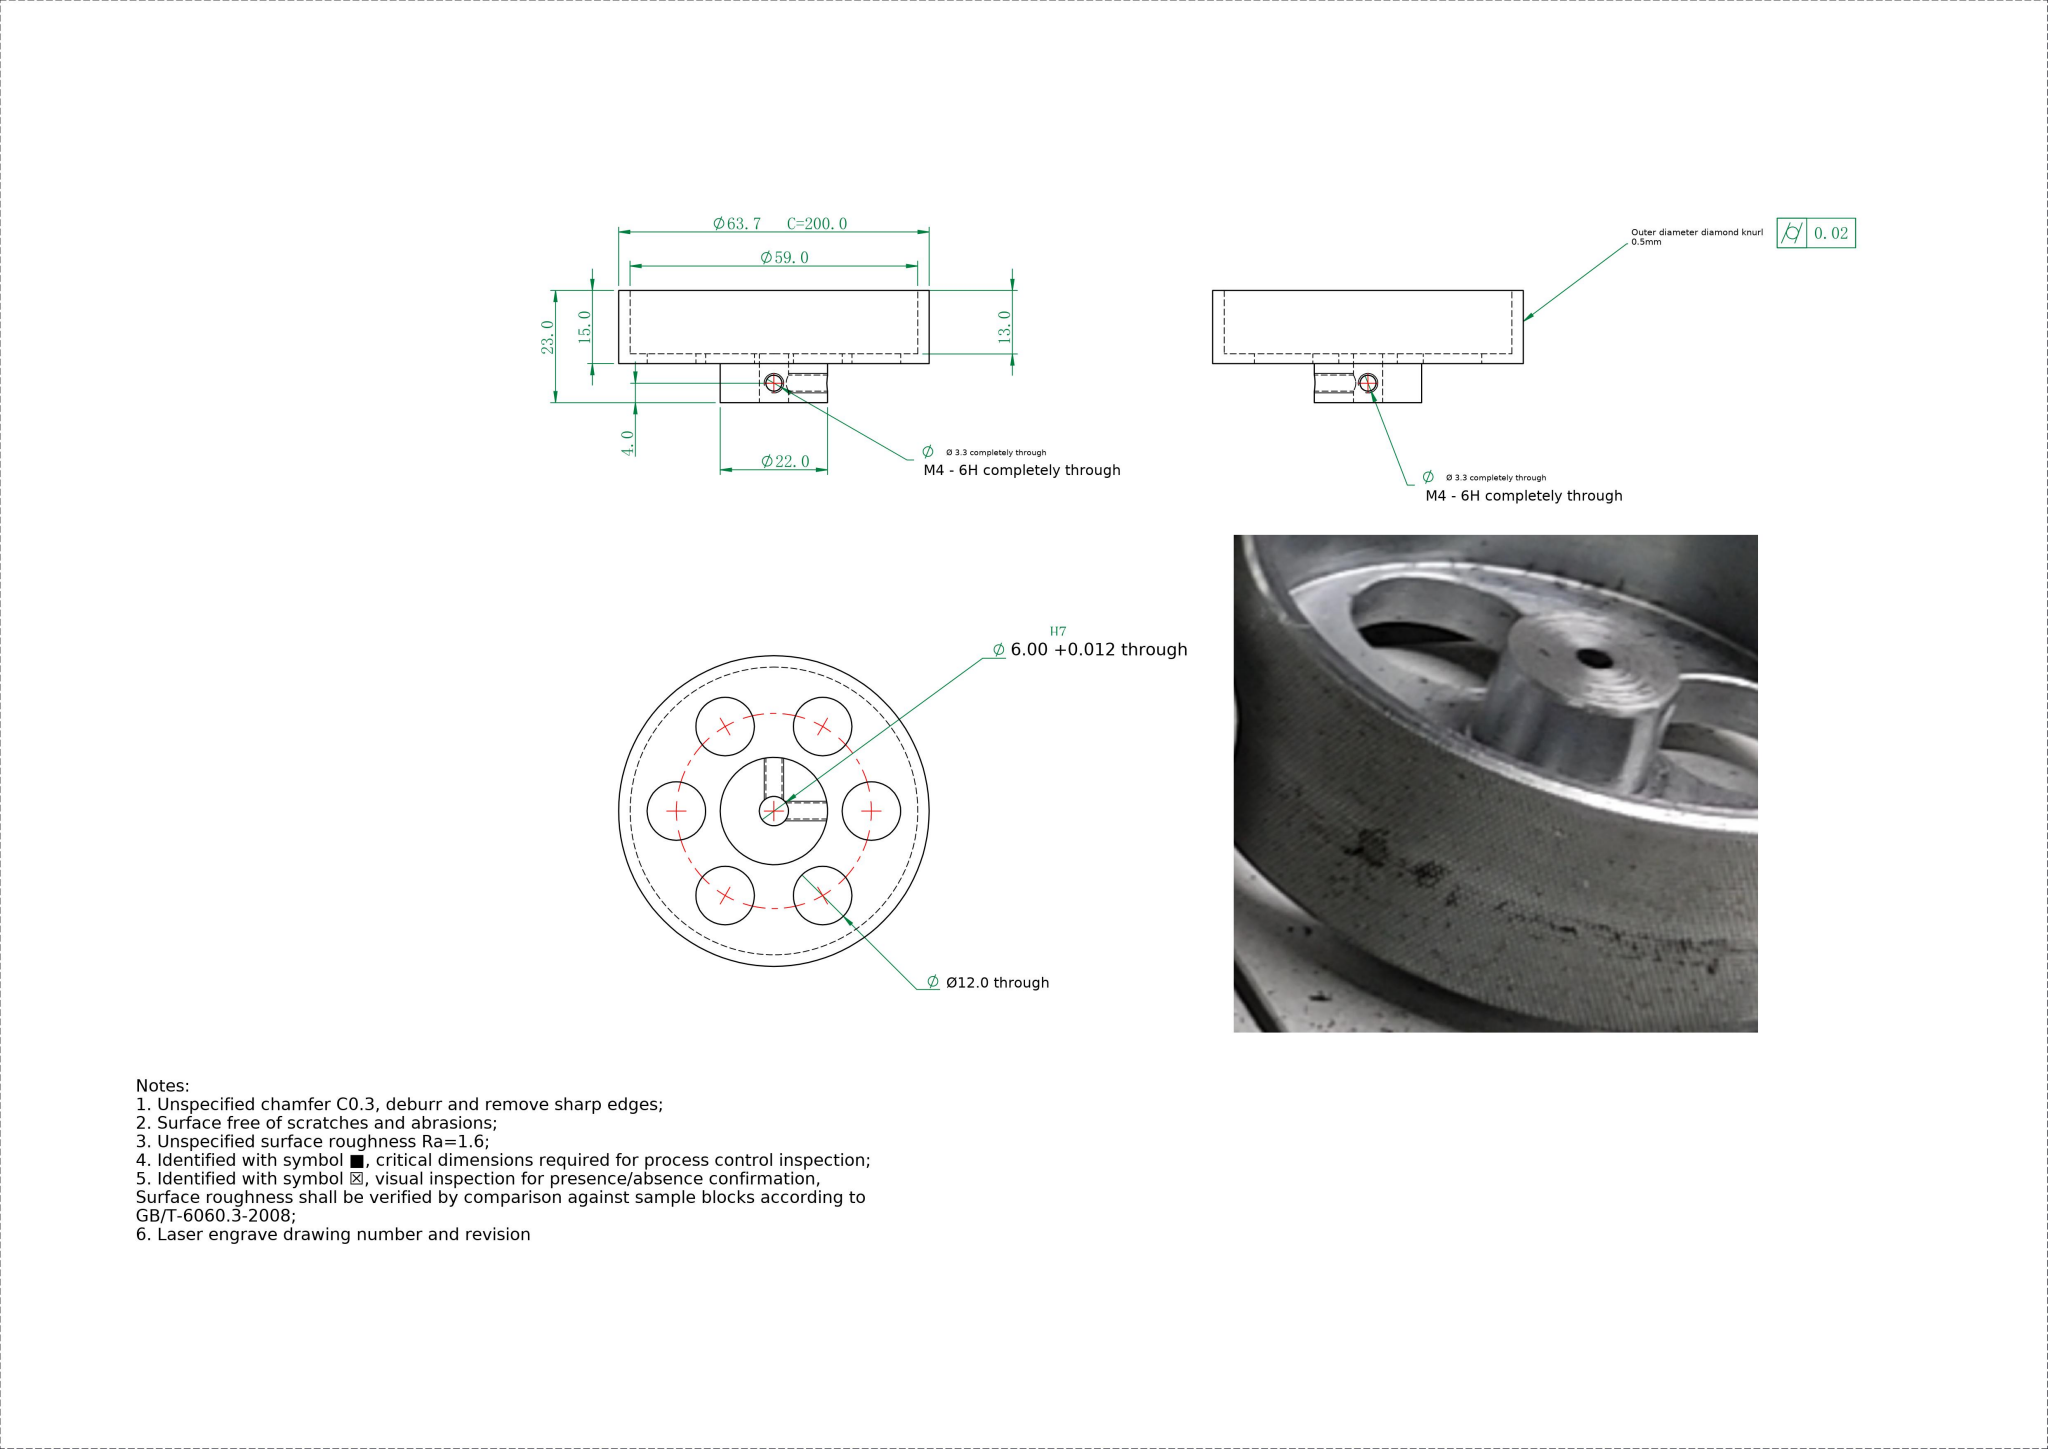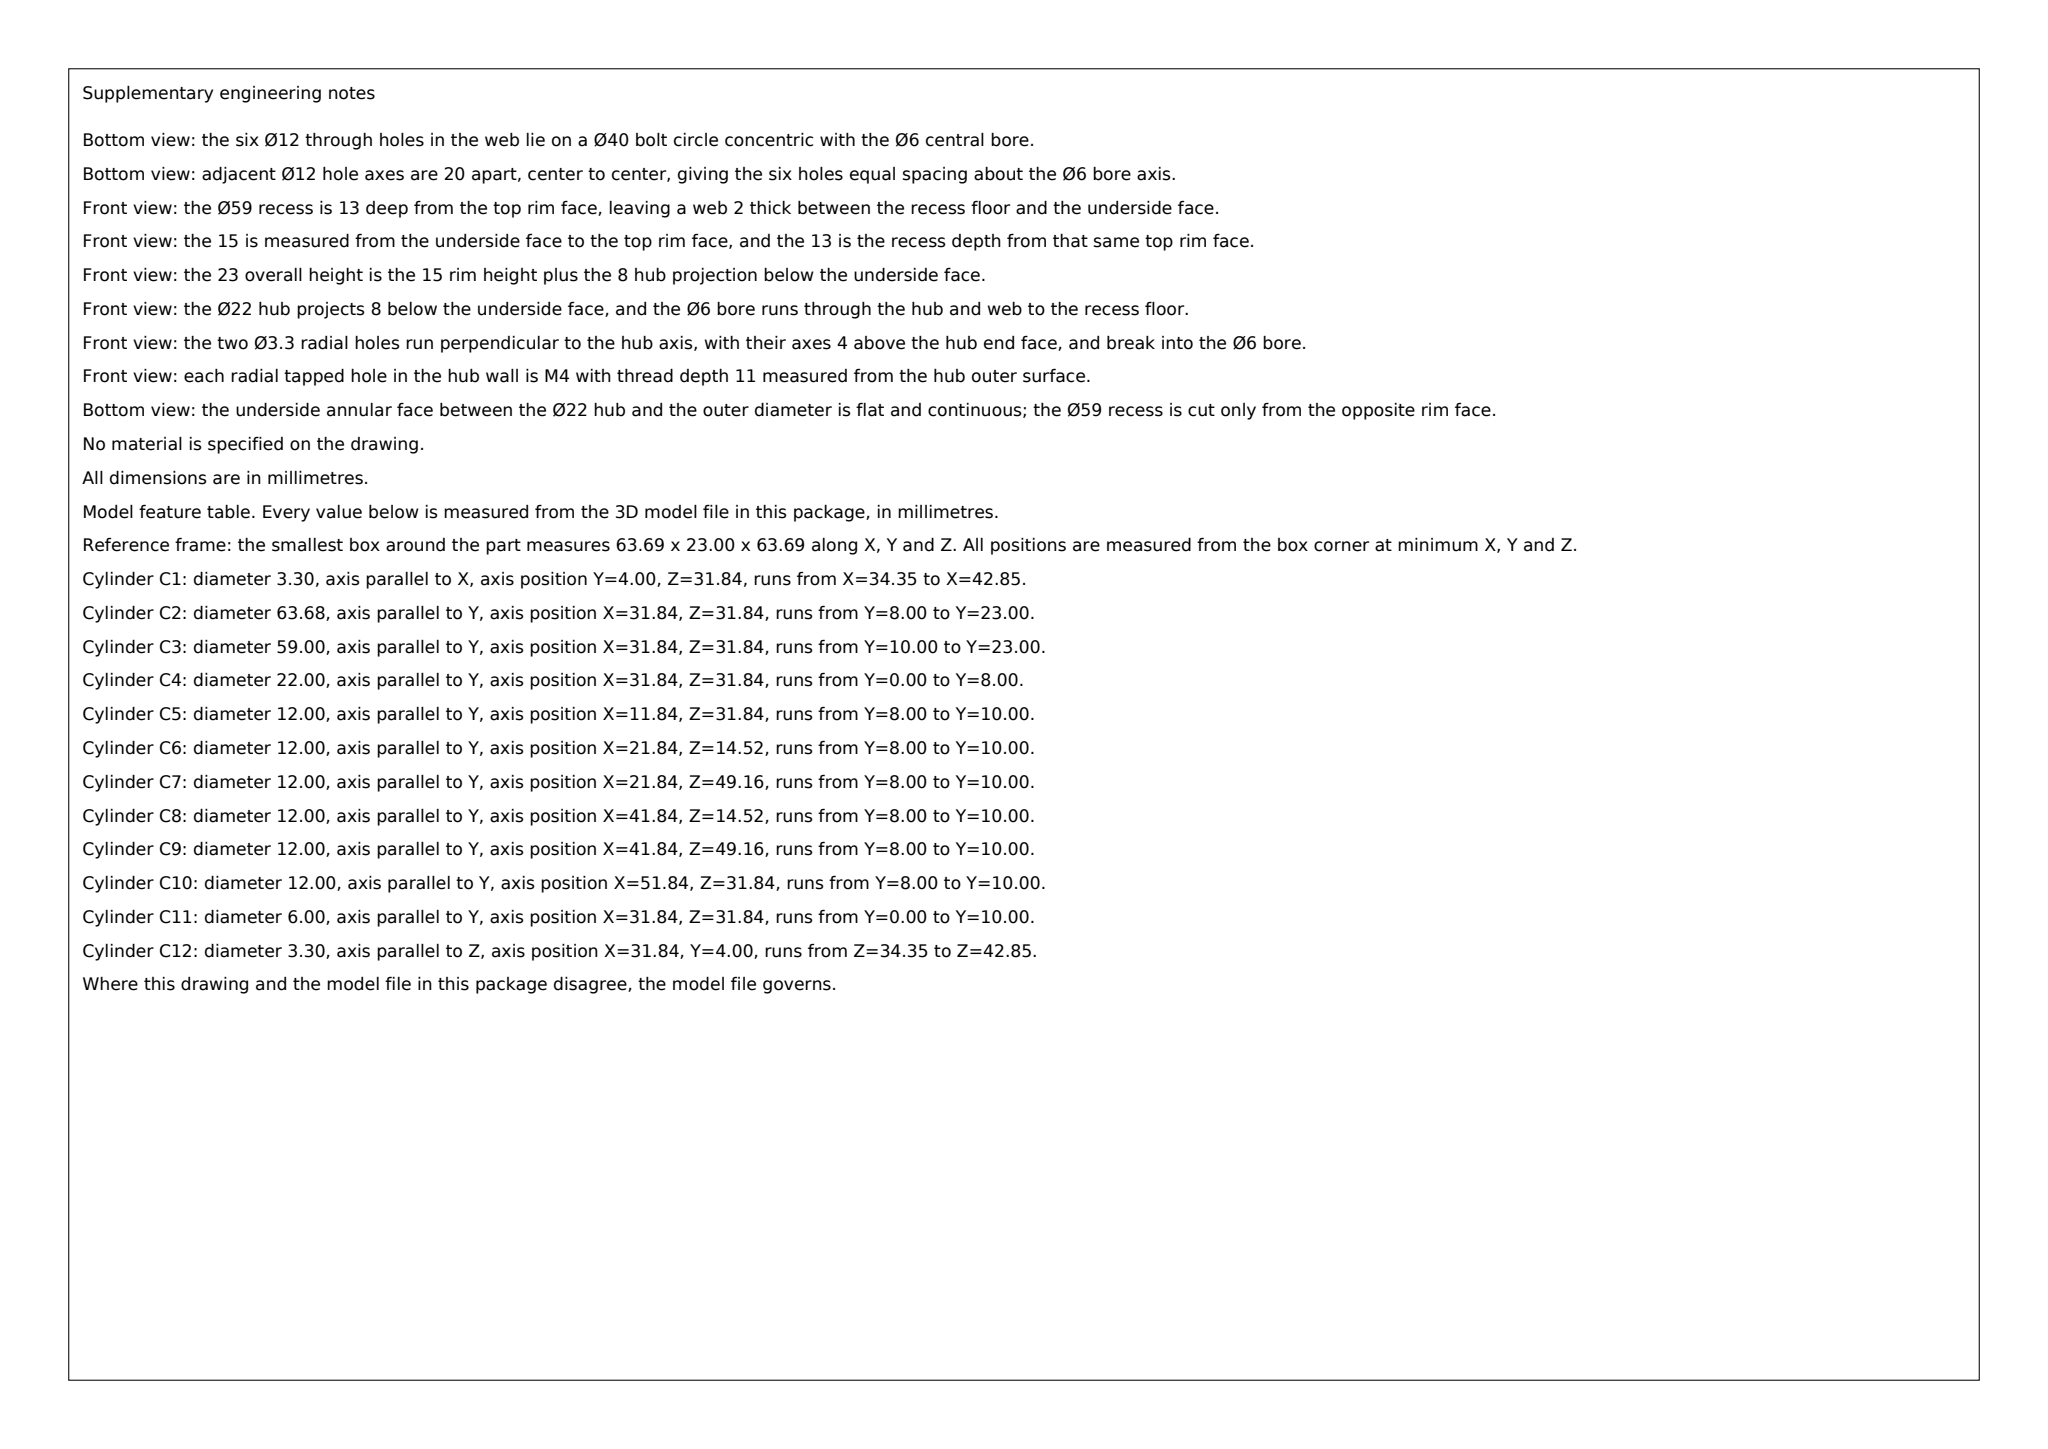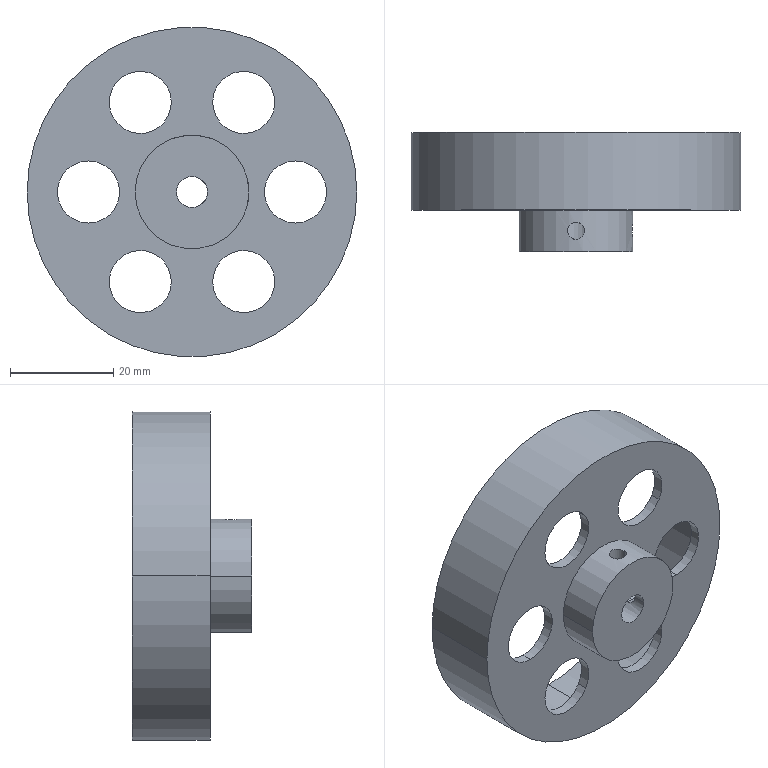Part | SolidWorks | mm | 1 solid | 28 faces | box 63.69 x 23 x 63.69 mm | volume 13510 mm3 | cylinder 24 | plane 4 | commonest cylinder face diameters 12 x12 3.3 x4 6 x2 22 x2 59 x2 63.69 x2